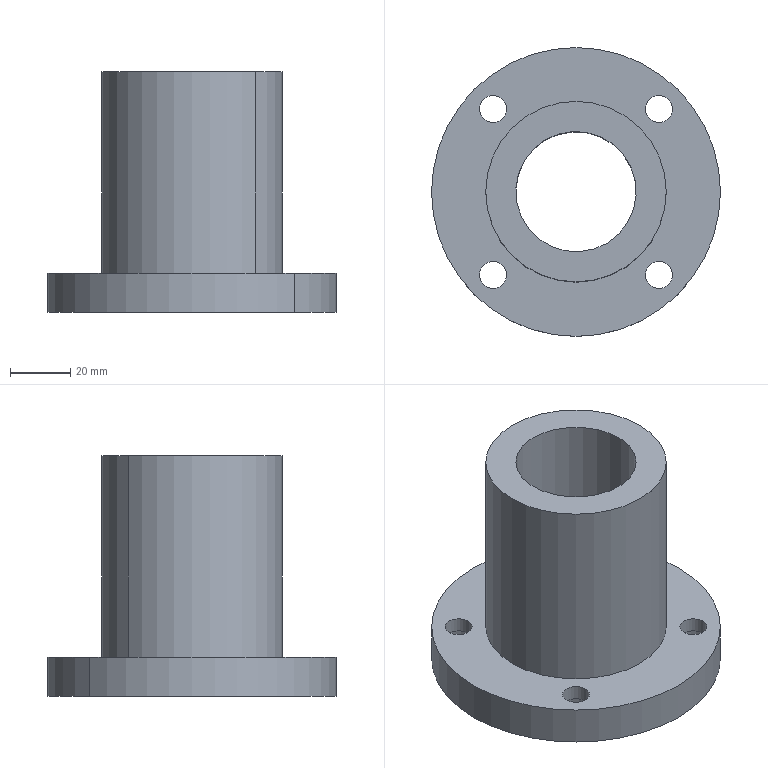Component | SolidWorks | LMF40UU-13 | 1 solid | 29 faces | box 96 x 96 x 80 mm | volume 176770 mm3 | cylinder 22 | plane 7 | commonest cylinder face diameters 9 x8 14 x8 96 x2 40 x2 60 x2 | material Standard Parts
STEP:
#1=CARTESIAN_POINT('',(7.771,5.019,-18.07));
#2=VERTEX_POINT('',#1);
#3=CARTESIAN_POINT('',(7.521,5.269,-18.07));
#4=VERTEX_POINT('',#3);
#5=CARTESIAN_POINT('',(7.646,5.144,-18.07));
#6=DIRECTION('',(0.,0.,-1.));
#7=DIRECTION('',(-0.7071,0.7071,0.));
#8=AXIS2_PLACEMENT_3D('',#5,#6,#7);
#9=CIRCLE('',#8,0.1772);
#10=EDGE_CURVE('',#2,#4,#9,.T.);
#11=ORIENTED_EDGE('',*,*,#10,.F.);
#12=CARTESIAN_POINT('',(7.771,5.019,-18.262));
#13=VERTEX_POINT('',#12);
#14=CARTESIAN_POINT('',(7.771,5.019,-18.262));
#15=DIRECTION('',(0.,0.,-1.));
#16=VECTOR('',#15,39.37);
#17=LINE('',#14,#16);
#18=EDGE_CURVE('',#2,#13,#17,.T.);
#19=ORIENTED_EDGE('',*,*,#18,.T.);
#20=CARTESIAN_POINT('',(7.521,5.269,-18.262));
#21=VERTEX_POINT('',#20);
#22=CARTESIAN_POINT('',(7.646,5.144,-18.262));
#23=DIRECTION('',(0.,0.,-1.));
#24=DIRECTION('',(-0.7071,0.7071,0.));
#25=AXIS2_PLACEMENT_3D('',#22,#23,#24);
#26=CIRCLE('',#25,0.1772);
#27=EDGE_CURVE('',#13,#21,#26,.T.);
#28=ORIENTED_EDGE('',*,*,#27,.T.);
#29=CARTESIAN_POINT('',(7.521,5.269,-18.262));
#30=DIRECTION('',(0.,0.,-1.));
#31=VECTOR('',#30,39.37);
#32=LINE('',#29,#31);
#33=EDGE_CURVE('',#4,#21,#32,.T.);
#34=ORIENTED_EDGE('',*,*,#33,.F.);
#35=EDGE_LOOP('',(#11,#19,#28,#34));
#36=FACE_OUTER_BOUND('',#35,.T.);
#37=CARTESIAN_POINT('',(7.646,5.144,-18.262));
#38=DIRECTION('',(0.,0.,-1.));
#39=DIRECTION('',(-0.7071,0.7071,0.));
#40=AXIS2_PLACEMENT_3D('',#37,#38,#39);
#41=CYLINDRICAL_SURFACE('',#40,0.1772);
#42=ADVANCED_FACE('',(#36),#41,.F.);
#43=CARTESIAN_POINT('',(7.771,2.847,-18.07));
#44=VERTEX_POINT('',#43);
#45=CARTESIAN_POINT('',(7.521,3.098,-18.07));
#46=VERTEX_POINT('',#45);
#47=CARTESIAN_POINT('',(7.646,2.973,-18.07));
#48=DIRECTION('',(0.,0.,-1.));
#49=DIRECTION('',(-0.7071,0.7071,0.));
#50=AXIS2_PLACEMENT_3D('',#47,#48,#49);
#51=CIRCLE('',#50,0.1772);
#52=EDGE_CURVE('',#44,#46,#51,.T.);
#53=ORIENTED_EDGE('',*,*,#52,.F.);
#54=CARTESIAN_POINT('',(7.771,2.847,-18.262));
#55=VERTEX_POINT('',#54);
#56=CARTESIAN_POINT('',(7.771,2.847,-18.262));
#57=DIRECTION('',(0.,0.,-1.));
#58=VECTOR('',#57,39.37);
#59=LINE('',#56,#58);
#60=EDGE_CURVE('',#44,#55,#59,.T.);
#61=ORIENTED_EDGE('',*,*,#60,.T.);
#62=CARTESIAN_POINT('',(7.521,3.098,-18.262));
#63=VERTEX_POINT('',#62);
#64=CARTESIAN_POINT('',(7.646,2.973,-18.262));
#65=DIRECTION('',(0.,0.,-1.));
#66=DIRECTION('',(-0.7071,0.7071,0.));
#67=AXIS2_PLACEMENT_3D('',#64,#65,#66);
#68=CIRCLE('',#67,0.1772);
#69=EDGE_CURVE('',#55,#63,#68,.T.);
#70=ORIENTED_EDGE('',*,*,#69,.T.);
#71=CARTESIAN_POINT('',(7.521,3.098,-18.262));
#72=DIRECTION('',(0.,0.,-1.));
#73=VECTOR('',#72,39.37);
#74=LINE('',#71,#73);
#75=EDGE_CURVE('',#46,#63,#74,.T.);
#76=ORIENTED_EDGE('',*,*,#75,.F.);
#77=EDGE_LOOP('',(#53,#61,#70,#76));
#78=FACE_OUTER_BOUND('',#77,.T.);
#79=CARTESIAN_POINT('',(7.646,2.973,-18.262));
#80=DIRECTION('',(0.,0.,-1.));
#81=DIRECTION('',(-0.7071,0.7071,0.));
#82=AXIS2_PLACEMENT_3D('',#79,#80,#81);
#83=CYLINDRICAL_SURFACE('',#82,0.1772);
#84=ADVANCED_FACE('',(#78),#83,.F.);
#85=CARTESIAN_POINT('',(9.943,2.847,-18.07));
#86=VERTEX_POINT('',#85);
#87=CARTESIAN_POINT('',(9.692,3.098,-18.07));
#88=VERTEX_POINT('',#87);
#89=CARTESIAN_POINT('',(9.817,2.973,-18.07));
#90=DIRECTION('',(0.,0.,-1.));
#91=DIRECTION('',(-0.7071,0.7071,0.));
#92=AXIS2_PLACEMENT_3D('',#89,#90,#91);
#93=CIRCLE('',#92,0.1772);
#94=EDGE_CURVE('',#86,#88,#93,.T.);
#95=ORIENTED_EDGE('',*,*,#94,.F.);
#96=CARTESIAN_POINT('',(9.943,2.847,-18.262));
#97=VERTEX_POINT('',#96);
#98=CARTESIAN_POINT('',(9.943,2.847,-18.262));
#99=DIRECTION('',(0.,0.,-1.));
#100=VECTOR('',#99,39.37);
#101=LINE('',#98,#100);
#102=EDGE_CURVE('',#86,#97,#101,.T.);
#103=ORIENTED_EDGE('',*,*,#102,.T.);
#104=CARTESIAN_POINT('',(9.692,3.098,-18.262));
#105=VERTEX_POINT('',#104);
#106=CARTESIAN_POINT('',(9.817,2.973,-18.262));
#107=DIRECTION('',(0.,0.,-1.));
#108=DIRECTION('',(-0.7071,0.7071,0.));
#109=AXIS2_PLACEMENT_3D('',#106,#107,#108);
#110=CIRCLE('',#109,0.1772);
#111=EDGE_CURVE('',#97,#105,#110,.T.);
#112=ORIENTED_EDGE('',*,*,#111,.T.);
#113=CARTESIAN_POINT('',(9.692,3.098,-18.262));
#114=DIRECTION('',(0.,0.,-1.));
#115=VECTOR('',#114,39.37);
#116=LINE('',#113,#115);
#117=EDGE_CURVE('',#88,#105,#116,.T.);
#118=ORIENTED_EDGE('',*,*,#117,.F.);
#119=EDGE_LOOP('',(#95,#103,#112,#118));
#120=FACE_OUTER_BOUND('',#119,.T.);
#121=CARTESIAN_POINT('',(9.817,2.973,-18.262));
#122=DIRECTION('',(0.,0.,-1.));
#123=DIRECTION('',(-0.7071,0.7071,0.));
#124=AXIS2_PLACEMENT_3D('',#121,#122,#123);
#125=CYLINDRICAL_SURFACE('',#124,0.1772);
#126=ADVANCED_FACE('',(#120),#125,.F.);
#127=CARTESIAN_POINT('',(7.841,4.949,-18.262));
#128=VERTEX_POINT('',#127);
#129=CARTESIAN_POINT('',(7.451,5.339,-18.262));
#130=VERTEX_POINT('',#129);
#131=CARTESIAN_POINT('',(7.646,5.144,-18.262));
#132=DIRECTION('',(0.,0.,-1.));
#133=DIRECTION('',(-0.7071,0.7071,0.));
#134=AXIS2_PLACEMENT_3D('',#131,#132,#133);
#135=CIRCLE('',#134,0.2756);
#136=EDGE_CURVE('',#128,#130,#135,.T.);
#137=ORIENTED_EDGE('',*,*,#136,.F.);
#138=CARTESIAN_POINT('',(7.841,4.949,-18.581));
#139=VERTEX_POINT('',#138);
#140=CARTESIAN_POINT('',(7.841,4.949,-18.581));
#141=DIRECTION('',(0.,0.,-1.));
#142=VECTOR('',#141,39.37);
#143=LINE('',#140,#142);
#144=EDGE_CURVE('',#128,#139,#143,.T.);
#145=ORIENTED_EDGE('',*,*,#144,.T.);
#146=CARTESIAN_POINT('',(7.451,5.339,-18.581));
#147=VERTEX_POINT('',#146);
#148=CARTESIAN_POINT('',(7.646,5.144,-18.581));
#149=DIRECTION('',(0.,0.,-1.));
#150=DIRECTION('',(-0.7071,0.7071,0.));
#151=AXIS2_PLACEMENT_3D('',#148,#149,#150);
#152=CIRCLE('',#151,0.2756);
#153=EDGE_CURVE('',#139,#147,#152,.T.);
#154=ORIENTED_EDGE('',*,*,#153,.T.);
#155=CARTESIAN_POINT('',(7.451,5.339,-18.581));
#156=DIRECTION('',(0.,0.,-1.));
#157=VECTOR('',#156,39.37);
#158=LINE('',#155,#157);
#159=EDGE_CURVE('',#130,#147,#158,.T.);
#160=ORIENTED_EDGE('',*,*,#159,.F.);
#161=EDGE_LOOP('',(#137,#145,#154,#160));
#162=FACE_OUTER_BOUND('',#161,.T.);
#163=CARTESIAN_POINT('',(7.646,5.144,-18.581));
#164=DIRECTION('',(0.,0.,-1.));
#165=DIRECTION('',(-0.7071,0.7071,0.));
#166=AXIS2_PLACEMENT_3D('',#163,#164,#165);
#167=CYLINDRICAL_SURFACE('',#166,0.2756);
#168=ADVANCED_FACE('',(#162),#167,.F.);
#169=CARTESIAN_POINT('',(7.841,2.778,-18.262));
#170=VERTEX_POINT('',#169);
#171=CARTESIAN_POINT('',(7.451,3.168,-18.262));
#172=VERTEX_POINT('',#171);
#173=CARTESIAN_POINT('',(7.646,2.973,-18.262));
#174=DIRECTION('',(0.,0.,-1.));
#175=DIRECTION('',(-0.7071,0.7071,0.));
#176=AXIS2_PLACEMENT_3D('',#173,#174,#175);
#177=CIRCLE('',#176,0.2756);
#178=EDGE_CURVE('',#170,#172,#177,.T.);
#179=ORIENTED_EDGE('',*,*,#178,.F.);
#180=CARTESIAN_POINT('',(7.841,2.778,-18.581));
#181=VERTEX_POINT('',#180);
#182=CARTESIAN_POINT('',(7.841,2.778,-18.581));
#183=DIRECTION('',(0.,0.,-1.));
#184=VECTOR('',#183,39.37);
#185=LINE('',#182,#184);
#186=EDGE_CURVE('',#170,#181,#185,.T.);
#187=ORIENTED_EDGE('',*,*,#186,.T.);
#188=CARTESIAN_POINT('',(7.451,3.168,-18.581));
#189=VERTEX_POINT('',#188);
#190=CARTESIAN_POINT('',(7.646,2.973,-18.581));
#191=DIRECTION('',(0.,0.,-1.));
#192=DIRECTION('',(-0.7071,0.7071,0.));
#193=AXIS2_PLACEMENT_3D('',#190,#191,#192);
#194=CIRCLE('',#193,0.2756);
#195=EDGE_CURVE('',#181,#189,#194,.T.);
#196=ORIENTED_EDGE('',*,*,#195,.T.);
#197=CARTESIAN_POINT('',(7.451,3.168,-18.581));
#198=DIRECTION('',(0.,0.,-1.));
#199=VECTOR('',#198,39.37);
#200=LINE('',#197,#199);
#201=EDGE_CURVE('',#172,#189,#200,.T.);
#202=ORIENTED_EDGE('',*,*,#201,.F.);
#203=EDGE_LOOP('',(#179,#187,#196,#202));
#204=FACE_OUTER_BOUND('',#203,.T.);
#205=CARTESIAN_POINT('',(7.646,2.973,-18.581));
#206=DIRECTION('',(0.,0.,-1.));
#207=DIRECTION('',(-0.7071,0.7071,0.));
#208=AXIS2_PLACEMENT_3D('',#205,#206,#207);
#209=CYLINDRICAL_SURFACE('',#208,0.2756);
#210=ADVANCED_FACE('',(#204),#209,.F.);
#211=CARTESIAN_POINT('',(10.012,2.778,-18.262));
#212=VERTEX_POINT('',#211);
#213=CARTESIAN_POINT('',(9.623,3.168,-18.262));
#214=VERTEX_POINT('',#213);
#215=CARTESIAN_POINT('',(9.817,2.973,-18.262));
#216=DIRECTION('',(0.,0.,-1.));
#217=DIRECTION('',(-0.7071,0.7071,0.));
#218=AXIS2_PLACEMENT_3D('',#215,#216,#217);
#219=CIRCLE('',#218,0.2756);
#220=EDGE_CURVE('',#212,#214,#219,.T.);
#221=ORIENTED_EDGE('',*,*,#220,.F.);
#222=CARTESIAN_POINT('',(10.012,2.778,-18.581));
#223=VERTEX_POINT('',#222);
#224=CARTESIAN_POINT('',(10.012,2.778,-18.581));
#225=DIRECTION('',(0.,0.,-1.));
#226=VECTOR('',#225,39.37);
#227=LINE('',#224,#226);
#228=EDGE_CURVE('',#212,#223,#227,.T.);
#229=ORIENTED_EDGE('',*,*,#228,.T.);
#230=CARTESIAN_POINT('',(9.623,3.168,-18.581));
#231=VERTEX_POINT('',#230);
#232=CARTESIAN_POINT('',(9.817,2.973,-18.581));
#233=DIRECTION('',(0.,0.,-1.));
#234=DIRECTION('',(-0.7071,0.7071,0.));
#235=AXIS2_PLACEMENT_3D('',#232,#233,#234);
#236=CIRCLE('',#235,0.2756);
#237=EDGE_CURVE('',#223,#231,#236,.T.);
#238=ORIENTED_EDGE('',*,*,#237,.T.);
#239=CARTESIAN_POINT('',(9.623,3.168,-18.581));
#240=DIRECTION('',(0.,0.,-1.));
#241=VECTOR('',#240,39.37);
#242=LINE('',#239,#241);
#243=EDGE_CURVE('',#214,#231,#242,.T.);
#244=ORIENTED_EDGE('',*,*,#243,.F.);
#245=EDGE_LOOP('',(#221,#229,#238,#244));
#246=FACE_OUTER_BOUND('',#245,.T.);
#247=CARTESIAN_POINT('',(9.817,2.973,-18.581));
#248=DIRECTION('',(0.,0.,-1.));
#249=DIRECTION('',(-0.7071,0.7071,0.));
#250=AXIS2_PLACEMENT_3D('',#247,#248,#249);
#251=CYLINDRICAL_SURFACE('',#250,0.2756);
#252=ADVANCED_FACE('',(#246),#251,.F.);
#253=CARTESIAN_POINT('',(9.943,5.019,-18.07));
#254=VERTEX_POINT('',#253);
#255=CARTESIAN_POINT('',(9.692,5.269,-18.07));
#256=VERTEX_POINT('',#255);
#257=CARTESIAN_POINT('',(9.817,5.144,-18.07));
#258=DIRECTION('',(0.,0.,-1.));
#259=DIRECTION('',(-0.7071,0.7071,0.));
#260=AXIS2_PLACEMENT_3D('',#257,#258,#259);
#261=CIRCLE('',#260,0.1772);
#262=EDGE_CURVE('',#254,#256,#261,.T.);
#263=ORIENTED_EDGE('',*,*,#262,.F.);
#264=CARTESIAN_POINT('',(9.943,5.019,-18.262));
#265=VERTEX_POINT('',#264);
#266=CARTESIAN_POINT('',(9.943,5.019,-18.262));
#267=DIRECTION('',(0.,0.,-1.));
#268=VECTOR('',#267,39.37);
#269=LINE('',#266,#268);
#270=EDGE_CURVE('',#254,#265,#269,.T.);
#271=ORIENTED_EDGE('',*,*,#270,.T.);
#272=CARTESIAN_POINT('',(9.692,5.269,-18.262));
#273=VERTEX_POINT('',#272);
#274=CARTESIAN_POINT('',(9.817,5.144,-18.262));
#275=DIRECTION('',(0.,0.,-1.));
#276=DIRECTION('',(-0.7071,0.7071,0.));
#277=AXIS2_PLACEMENT_3D('',#274,#275,#276);
#278=CIRCLE('',#277,0.1772);
#279=EDGE_CURVE('',#265,#273,#278,.T.);
#280=ORIENTED_EDGE('',*,*,#279,.T.);
#281=CARTESIAN_POINT('',(9.692,5.269,-18.262));
#282=DIRECTION('',(0.,0.,-1.));
#283=VECTOR('',#282,39.37);
#284=LINE('',#281,#283);
#285=EDGE_CURVE('',#256,#273,#284,.T.);
#286=ORIENTED_EDGE('',*,*,#285,.F.);
#287=EDGE_LOOP('',(#263,#271,#280,#286));
#288=FACE_OUTER_BOUND('',#287,.T.);
#289=CARTESIAN_POINT('',(9.817,5.144,-18.262));
#290=DIRECTION('',(0.,0.,-1.));
#291=DIRECTION('',(-0.7071,0.7071,0.));
#292=AXIS2_PLACEMENT_3D('',#289,#290,#291);
#293=CYLINDRICAL_SURFACE('',#292,0.1772);
#294=ADVANCED_FACE('',(#288),#293,.F.);
#295=CARTESIAN_POINT('',(10.012,4.949,-18.262));
#296=VERTEX_POINT('',#295);
#297=CARTESIAN_POINT('',(9.623,5.339,-18.262));
#298=VERTEX_POINT('',#297);
#299=CARTESIAN_POINT('',(9.817,5.144,-18.262));
#300=DIRECTION('',(0.,0.,-1.));
#301=DIRECTION('',(-0.7071,0.7071,0.));
#302=AXIS2_PLACEMENT_3D('',#299,#300,#301);
#303=CIRCLE('',#302,0.2756);
#304=EDGE_CURVE('',#296,#298,#303,.T.);
#305=ORIENTED_EDGE('',*,*,#304,.F.);
#306=CARTESIAN_POINT('',(10.012,4.949,-18.581));
#307=VERTEX_POINT('',#306);
#308=CARTESIAN_POINT('',(10.012,4.949,-18.581));
#309=DIRECTION('',(0.,0.,-1.));
#310=VECTOR('',#309,39.37);
#311=LINE('',#308,#310);
#312=EDGE_CURVE('',#296,#307,#311,.T.);
#313=ORIENTED_EDGE('',*,*,#312,.T.);
#314=CARTESIAN_POINT('',(9.623,5.339,-18.581));
#315=VERTEX_POINT('',#314);
#316=CARTESIAN_POINT('',(9.817,5.144,-18.581));
#317=DIRECTION('',(0.,0.,-1.));
#318=DIRECTION('',(-0.7071,0.7071,0.));
#319=AXIS2_PLACEMENT_3D('',#316,#317,#318);
#320=CIRCLE('',#319,0.2756);
#321=EDGE_CURVE('',#307,#315,#320,.T.);
#322=ORIENTED_EDGE('',*,*,#321,.T.);
#323=CARTESIAN_POINT('',(9.623,5.339,-18.581));
#324=DIRECTION('',(0.,0.,-1.));
#325=VECTOR('',#324,39.37);
#326=LINE('',#323,#325);
#327=EDGE_CURVE('',#298,#315,#326,.T.);
#328=ORIENTED_EDGE('',*,*,#327,.F.);
#329=EDGE_LOOP('',(#305,#313,#322,#328));
#330=FACE_OUTER_BOUND('',#329,.T.);
#331=CARTESIAN_POINT('',(9.817,5.144,-18.581));
#332=DIRECTION('',(0.,0.,-1.));
#333=DIRECTION('',(-0.7071,0.7071,0.));
#334=AXIS2_PLACEMENT_3D('',#331,#332,#333);
#335=CYLINDRICAL_SURFACE('',#334,0.2756);
#336=ADVANCED_FACE('',(#330),#335,.F.);
#337=CARTESIAN_POINT('',(7.395,5.395,-18.07));
#338=VERTEX_POINT('',#337);
#339=CARTESIAN_POINT('',(10.068,2.722,-18.07));
#340=VERTEX_POINT('',#339);
#341=CARTESIAN_POINT('',(8.732,4.058,-18.07));
#342=DIRECTION('',(0.,0.,-1.));
#343=DIRECTION('',(-0.7071,0.7071,0.));
#344=AXIS2_PLACEMENT_3D('',#341,#342,#343);
#345=CIRCLE('',#344,1.89);
#346=EDGE_CURVE('',#338,#340,#345,.T.);
#347=ORIENTED_EDGE('',*,*,#346,.T.);
#348=CARTESIAN_POINT('',(10.068,2.722,-18.581));
#349=VERTEX_POINT('',#348);
#350=CARTESIAN_POINT('',(10.068,2.722,-18.07));
#351=DIRECTION('',(0.,0.,-1.));
#352=VECTOR('',#351,39.37);
#353=LINE('',#350,#352);
#354=EDGE_CURVE('',#340,#349,#353,.T.);
#355=ORIENTED_EDGE('',*,*,#354,.T.);
#356=CARTESIAN_POINT('',(7.395,5.395,-18.581));
#357=VERTEX_POINT('',#356);
#358=CARTESIAN_POINT('',(8.732,4.058,-18.581));
#359=DIRECTION('',(0.,0.,-1.));
#360=DIRECTION('',(-0.7071,0.7071,0.));
#361=AXIS2_PLACEMENT_3D('',#358,#359,#360);
#362=CIRCLE('',#361,1.89);
#363=EDGE_CURVE('',#357,#349,#362,.T.);
#364=ORIENTED_EDGE('',*,*,#363,.F.);
#365=CARTESIAN_POINT('',(7.395,5.395,-18.07));
#366=DIRECTION('',(0.,0.,-1.));
#367=VECTOR('',#366,39.37);
#368=LINE('',#365,#367);
#369=EDGE_CURVE('',#338,#357,#368,.T.);
#370=ORIENTED_EDGE('',*,*,#369,.F.);
#371=EDGE_LOOP('',(#347,#355,#364,#370));
#372=FACE_OUTER_BOUND('',#371,.T.);
#373=CARTESIAN_POINT('',(8.732,4.058,-18.07));
#374=DIRECTION('',(0.,0.,-1.));
#375=DIRECTION('',(-0.7071,0.7071,0.));
#376=AXIS2_PLACEMENT_3D('',#373,#374,#375);
#377=CYLINDRICAL_SURFACE('',#376,1.89);
#378=ADVANCED_FACE('',(#372),#377,.T.);
#379=CARTESIAN_POINT('',(9.288,3.502,-15.432));
#380=VERTEX_POINT('',#379);
#381=CARTESIAN_POINT('',(8.175,4.615,-15.432));
#382=VERTEX_POINT('',#381);
#383=CARTESIAN_POINT('',(8.732,4.058,-15.432));
#384=DIRECTION('',(0.,0.,-1.));
#385=DIRECTION('',(-0.7071,0.7071,0.));
#386=AXIS2_PLACEMENT_3D('',#383,#384,#385);
#387=CIRCLE('',#386,0.7874);
#388=EDGE_CURVE('',#380,#382,#387,.T.);
#389=ORIENTED_EDGE('',*,*,#388,.F.);
#390=CARTESIAN_POINT('',(9.288,3.502,-18.581));
#391=VERTEX_POINT('',#390);
#392=CARTESIAN_POINT('',(9.288,3.502,-15.432));
#393=DIRECTION('',(0.,0.,-1.));
#394=VECTOR('',#393,39.37);
#395=LINE('',#392,#394);
#396=EDGE_CURVE('',#380,#391,#395,.T.);
#397=ORIENTED_EDGE('',*,*,#396,.T.);
#398=CARTESIAN_POINT('',(8.175,4.615,-18.581));
#399=VERTEX_POINT('',#398);
#400=CARTESIAN_POINT('',(8.732,4.058,-18.581));
#401=DIRECTION('',(0.,0.,-1.));
#402=DIRECTION('',(-0.7071,0.7071,0.));
#403=AXIS2_PLACEMENT_3D('',#400,#401,#402);
#404=CIRCLE('',#403,0.7874);
#405=EDGE_CURVE('',#391,#399,#404,.T.);
#406=ORIENTED_EDGE('',*,*,#405,.T.);
#407=CARTESIAN_POINT('',(8.175,4.615,-15.432));
#408=DIRECTION('',(0.,0.,-1.));
#409=VECTOR('',#408,39.37);
#410=LINE('',#407,#409);
#411=EDGE_CURVE('',#382,#399,#410,.T.);
#412=ORIENTED_EDGE('',*,*,#411,.F.);
#413=EDGE_LOOP('',(#389,#397,#406,#412));
#414=FACE_OUTER_BOUND('',#413,.T.);
#415=CARTESIAN_POINT('',(8.732,4.058,-15.432));
#416=DIRECTION('',(0.,0.,-1.));
#417=DIRECTION('',(-0.7071,0.7071,0.));
#418=AXIS2_PLACEMENT_3D('',#415,#416,#417);
#419=CYLINDRICAL_SURFACE('',#418,0.7874);
#420=ADVANCED_FACE('',(#414),#419,.F.);
#421=CARTESIAN_POINT('',(7.897,4.894,-15.432));
#422=VERTEX_POINT('',#421);
#423=CARTESIAN_POINT('',(9.567,3.223,-15.432));
#424=VERTEX_POINT('',#423);
#425=CARTESIAN_POINT('',(8.732,4.058,-15.432));
#426=DIRECTION('',(0.,0.,-1.));
#427=DIRECTION('',(-0.7071,0.7071,0.));
#428=AXIS2_PLACEMENT_3D('',#425,#426,#427);
#429=CIRCLE('',#428,1.181);
#430=EDGE_CURVE('',#422,#424,#429,.T.);
#431=ORIENTED_EDGE('',*,*,#430,.T.);
#432=CARTESIAN_POINT('',(9.567,3.223,-18.07));
#433=VERTEX_POINT('',#432);
#434=CARTESIAN_POINT('',(9.567,3.223,-15.432));
#435=DIRECTION('',(0.,0.,-1.));
#436=VECTOR('',#435,39.37);
#437=LINE('',#434,#436);
#438=EDGE_CURVE('',#424,#433,#437,.T.);
#439=ORIENTED_EDGE('',*,*,#438,.T.);
#440=CARTESIAN_POINT('',(7.897,4.894,-18.07));
#441=VERTEX_POINT('',#440);
#442=CARTESIAN_POINT('',(8.732,4.058,-18.07));
#443=DIRECTION('',(0.,0.,1.));
#444=DIRECTION('',(-0.7071,0.7071,0.));
#445=AXIS2_PLACEMENT_3D('',#442,#443,#444);
#446=CIRCLE('',#445,1.181);
#447=EDGE_CURVE('',#433,#441,#446,.T.);
#448=ORIENTED_EDGE('',*,*,#447,.T.);
#449=CARTESIAN_POINT('',(7.897,4.894,-15.432));
#450=DIRECTION('',(0.,0.,-1.));
#451=VECTOR('',#450,39.37);
#452=LINE('',#449,#451);
#453=EDGE_CURVE('',#422,#441,#452,.T.);
#454=ORIENTED_EDGE('',*,*,#453,.F.);
#455=EDGE_LOOP('',(#431,#439,#448,#454));
#456=FACE_OUTER_BOUND('',#455,.T.);
#457=CARTESIAN_POINT('',(8.732,4.058,-15.432));
#458=DIRECTION('',(0.,0.,-1.));
#459=DIRECTION('',(-0.7071,0.7071,0.));
#460=AXIS2_PLACEMENT_3D('',#457,#458,#459);
#461=CYLINDRICAL_SURFACE('',#460,1.181);
#462=ADVANCED_FACE('',(#456),#461,.T.);
#463=CARTESIAN_POINT('',(7.646,5.144,-18.262));
#464=DIRECTION('',(0.,0.,-1.));
#465=DIRECTION('',(-0.7071,0.7071,0.));
#466=AXIS2_PLACEMENT_3D('',#463,#464,#465);
#467=CIRCLE('',#466,0.2756);
#468=EDGE_CURVE('',#130,#128,#467,.T.);
#469=ORIENTED_EDGE('',*,*,#468,.T.);
#470=ORIENTED_EDGE('',*,*,#136,.T.);
#471=EDGE_LOOP('',(#469,#470));
#472=FACE_OUTER_BOUND('',#471,.T.);
#473=CARTESIAN_POINT('',(7.646,5.144,-18.262));
#474=DIRECTION('',(0.,0.,-1.));
#475=DIRECTION('',(-0.7071,0.7071,0.));
#476=AXIS2_PLACEMENT_3D('',#473,#474,#475);
#477=CIRCLE('',#476,0.1772);
#478=EDGE_CURVE('',#21,#13,#477,.T.);
#479=ORIENTED_EDGE('',*,*,#478,.F.);
#480=ORIENTED_EDGE('',*,*,#27,.F.);
#481=EDGE_LOOP('',(#479,#480));
#482=FACE_BOUND('',#481,.T.);
#483=CARTESIAN_POINT('',(7.646,5.144,-18.262));
#484=DIRECTION('',(0.,0.,1.));
#485=DIRECTION('',(0.7071,-0.7071,0.));
#486=AXIS2_PLACEMENT_3D('',#483,#484,#485);
#487=PLANE('',#486);
#488=ADVANCED_FACE('',(#472,#482),#487,.F.);
#489=CARTESIAN_POINT('',(7.646,2.973,-18.262));
#490=DIRECTION('',(0.,0.,-1.));
#491=DIRECTION('',(-0.7071,0.7071,0.));
#492=AXIS2_PLACEMENT_3D('',#489,#490,#491);
#493=CIRCLE('',#492,0.2756);
#494=EDGE_CURVE('',#172,#170,#493,.T.);
#495=ORIENTED_EDGE('',*,*,#494,.T.);
#496=ORIENTED_EDGE('',*,*,#178,.T.);
#497=EDGE_LOOP('',(#495,#496));
#498=FACE_OUTER_BOUND('',#497,.T.);
#499=CARTESIAN_POINT('',(7.646,2.973,-18.262));
#500=DIRECTION('',(0.,0.,-1.));
#501=DIRECTION('',(-0.7071,0.7071,0.));
#502=AXIS2_PLACEMENT_3D('',#499,#500,#501);
#503=CIRCLE('',#502,0.1772);
#504=EDGE_CURVE('',#63,#55,#503,.T.);
#505=ORIENTED_EDGE('',*,*,#504,.F.);
#506=ORIENTED_EDGE('',*,*,#69,.F.);
#507=EDGE_LOOP('',(#505,#506));
#508=FACE_BOUND('',#507,.T.);
#509=CARTESIAN_POINT('',(7.646,2.973,-18.262));
#510=DIRECTION('',(0.,0.,1.));
#511=DIRECTION('',(0.7071,-0.7071,0.));
#512=AXIS2_PLACEMENT_3D('',#509,#510,#511);
#513=PLANE('',#512);
#514=ADVANCED_FACE('',(#498,#508),#513,.F.);
#515=CARTESIAN_POINT('',(9.817,2.973,-18.262));
#516=DIRECTION('',(0.,0.,-1.));
#517=DIRECTION('',(-0.7071,0.7071,0.));
#518=AXIS2_PLACEMENT_3D('',#515,#516,#517);
#519=CIRCLE('',#518,0.2756);
#520=EDGE_CURVE('',#214,#212,#519,.T.);
#521=ORIENTED_EDGE('',*,*,#520,.T.);
#522=ORIENTED_EDGE('',*,*,#220,.T.);
#523=EDGE_LOOP('',(#521,#522));
#524=FACE_OUTER_BOUND('',#523,.T.);
#525=CARTESIAN_POINT('',(9.817,2.973,-18.262));
#526=DIRECTION('',(0.,0.,-1.));
#527=DIRECTION('',(-0.7071,0.7071,0.));
#528=AXIS2_PLACEMENT_3D('',#525,#526,#527);
#529=CIRCLE('',#528,0.1772);
#530=EDGE_CURVE('',#105,#97,#529,.T.);
#531=ORIENTED_EDGE('',*,*,#530,.F.);
#532=ORIENTED_EDGE('',*,*,#111,.F.);
#533=EDGE_LOOP('',(#531,#532));
#534=FACE_BOUND('',#533,.T.);
#535=CARTESIAN_POINT('',(9.817,2.973,-18.262));
#536=DIRECTION('',(0.,0.,1.));
#537=DIRECTION('',(0.7071,-0.7071,0.));
#538=AXIS2_PLACEMENT_3D('',#535,#536,#537);
#539=PLANE('',#538);
#540=ADVANCED_FACE('',(#524,#534),#539,.F.);
#541=CARTESIAN_POINT('',(9.817,5.144,-18.262));
#542=DIRECTION('',(0.,0.,-1.));
#543=DIRECTION('',(-0.7071,0.7071,0.));
#544=AXIS2_PLACEMENT_3D('',#541,#542,#543);
#545=CIRCLE('',#544,0.2756);
#546=EDGE_CURVE('',#298,#296,#545,.T.);
#547=ORIENTED_EDGE('',*,*,#546,.T.);
#548=ORIENTED_EDGE('',*,*,#304,.T.);
#549=EDGE_LOOP('',(#547,#548));
#550=FACE_OUTER_BOUND('',#549,.T.);
#551=CARTESIAN_POINT('',(9.817,5.144,-18.262));
#552=DIRECTION('',(0.,0.,-1.));
#553=DIRECTION('',(-0.7071,0.7071,0.));
#554=AXIS2_PLACEMENT_3D('',#551,#552,#553);
#555=CIRCLE('',#554,0.1772);
#556=EDGE_CURVE('',#273,#265,#555,.T.);
#557=ORIENTED_EDGE('',*,*,#556,.F.);
#558=ORIENTED_EDGE('',*,*,#279,.F.);
#559=EDGE_LOOP('',(#557,#558));
#560=FACE_BOUND('',#559,.T.);
#561=CARTESIAN_POINT('',(9.817,5.144,-18.262));
#562=DIRECTION('',(0.,0.,1.));
#563=DIRECTION('',(0.7071,-0.7071,0.));
#564=AXIS2_PLACEMENT_3D('',#561,#562,#563);
#565=PLANE('',#564);
#566=ADVANCED_FACE('',(#550,#560),#565,.F.);
#567=ORIENTED_EDGE('',*,*,#438,.F.);
#568=CARTESIAN_POINT('',(8.732,4.058,-15.432));
#569=DIRECTION('',(0.,0.,-1.));
#570=DIRECTION('',(-0.7071,0.7071,0.));
#571=AXIS2_PLACEMENT_3D('',#568,#569,#570);
#572=CIRCLE('',#571,1.181);
#573=EDGE_CURVE('',#424,#422,#572,.T.);
#574=ORIENTED_EDGE('',*,*,#573,.T.);
#575=ORIENTED_EDGE('',*,*,#453,.T.);
#576=CARTESIAN_POINT('',(8.732,4.058,-18.07));
#577=DIRECTION('',(0.,0.,1.));
#578=DIRECTION('',(-0.7071,0.7071,0.));
#579=AXIS2_PLACEMENT_3D('',#576,#577,#578);
#580=CIRCLE('',#579,1.181);
#581=EDGE_CURVE('',#441,#433,#580,.T.);
#582=ORIENTED_EDGE('',*,*,#581,.T.);
#583=EDGE_LOOP('',(#567,#574,#575,#582));
#584=FACE_OUTER_BOUND('',#583,.T.);
#585=CARTESIAN_POINT('',(8.732,4.058,-15.432));
#586=DIRECTION('',(0.,0.,-1.));
#587=DIRECTION('',(-0.7071,0.7071,0.));
#588=AXIS2_PLACEMENT_3D('',#585,#586,#587);
#589=CYLINDRICAL_SURFACE('',#588,1.181);
#590=ADVANCED_FACE('',(#584),#589,.T.);
#591=CARTESIAN_POINT('',(8.732,4.058,-15.432));
#592=DIRECTION('',(0.,0.,-1.));
#593=DIRECTION('',(-0.7071,0.7071,0.));
#594=AXIS2_PLACEMENT_3D('',#591,#592,#593);
#595=CIRCLE('',#594,0.7874);
#596=EDGE_CURVE('',#382,#380,#595,.T.);
#597=ORIENTED_EDGE('',*,*,#596,.T.);
#598=ORIENTED_EDGE('',*,*,#388,.T.);
#599=EDGE_LOOP('',(#597,#598));
#600=FACE_BOUND('',#599,.T.);
#601=ORIENTED_EDGE('',*,*,#430,.F.);
#602=ORIENTED_EDGE('',*,*,#573,.F.);
#603=EDGE_LOOP('',(#601,#602));
#604=FACE_OUTER_BOUND('',#603,.T.);
#605=CARTESIAN_POINT('',(8.732,4.058,-15.432));
#606=DIRECTION('',(0.,0.,-1.));
#607=DIRECTION('',(-0.7071,0.7071,0.));
#608=AXIS2_PLACEMENT_3D('',#605,#606,#607);
#609=PLANE('',#608);
#610=ADVANCED_FACE('',(#600,#604),#609,.F.);
#611=ORIENTED_EDGE('',*,*,#396,.F.);
#612=ORIENTED_EDGE('',*,*,#596,.F.);
#613=ORIENTED_EDGE('',*,*,#411,.T.);
#614=CARTESIAN_POINT('',(8.732,4.058,-18.581));
#615=DIRECTION('',(0.,0.,-1.));
#616=DIRECTION('',(-0.7071,0.7071,0.));
#617=AXIS2_PLACEMENT_3D('',#614,#615,#616);
#618=CIRCLE('',#617,0.7874);
#619=EDGE_CURVE('',#399,#391,#618,.T.);
#620=ORIENTED_EDGE('',*,*,#619,.T.);
#621=EDGE_LOOP('',(#611,#612,#613,#620));
#622=FACE_OUTER_BOUND('',#621,.T.);
#623=CARTESIAN_POINT('',(8.732,4.058,-15.432));
#624=DIRECTION('',(0.,0.,-1.));
#625=DIRECTION('',(-0.7071,0.7071,0.));
#626=AXIS2_PLACEMENT_3D('',#623,#624,#625);
#627=CYLINDRICAL_SURFACE('',#626,0.7874);
#628=ADVANCED_FACE('',(#622),#627,.F.);
#629=CARTESIAN_POINT('',(7.646,5.144,-18.581));
#630=DIRECTION('',(0.,0.,-1.));
#631=DIRECTION('',(-0.7071,0.7071,0.));
#632=AXIS2_PLACEMENT_3D('',#629,#630,#631);
#633=CIRCLE('',#632,0.2756);
#634=EDGE_CURVE('',#147,#139,#633,.T.);
#635=ORIENTED_EDGE('',*,*,#634,.F.);
#636=ORIENTED_EDGE('',*,*,#153,.F.);
#637=EDGE_LOOP('',(#635,#636));
#638=FACE_BOUND('',#637,.T.);
#639=CARTESIAN_POINT('',(7.646,2.973,-18.581));
#640=DIRECTION('',(0.,0.,-1.));
#641=DIRECTION('',(-0.7071,0.7071,0.));
#642=AXIS2_PLACEMENT_3D('',#639,#640,#641);
#643=CIRCLE('',#642,0.2756);
#644=EDGE_CURVE('',#189,#181,#643,.T.);
#645=ORIENTED_EDGE('',*,*,#644,.F.);
#646=ORIENTED_EDGE('',*,*,#195,.F.);
#647=EDGE_LOOP('',(#645,#646));
#648=FACE_BOUND('',#647,.T.);
#649=CARTESIAN_POINT('',(9.817,2.973,-18.581));
#650=DIRECTION('',(0.,0.,-1.));
#651=DIRECTION('',(-0.7071,0.7071,0.));
#652=AXIS2_PLACEMENT_3D('',#649,#650,#651);
#653=CIRCLE('',#652,0.2756);
#654=EDGE_CURVE('',#231,#223,#653,.T.);
#655=ORIENTED_EDGE('',*,*,#654,.F.);
#656=ORIENTED_EDGE('',*,*,#237,.F.);
#657=EDGE_LOOP('',(#655,#656));
#658=FACE_BOUND('',#657,.T.);
#659=CARTESIAN_POINT('',(9.817,5.144,-18.581));
#660=DIRECTION('',(0.,0.,-1.));
#661=DIRECTION('',(-0.7071,0.7071,0.));
#662=AXIS2_PLACEMENT_3D('',#659,#660,#661);
#663=CIRCLE('',#662,0.2756);
#664=EDGE_CURVE('',#315,#307,#663,.T.);
#665=ORIENTED_EDGE('',*,*,#664,.F.);
#666=ORIENTED_EDGE('',*,*,#321,.F.);
#667=EDGE_LOOP('',(#665,#666));
#668=FACE_BOUND('',#667,.T.);
#669=ORIENTED_EDGE('',*,*,#619,.F.);
#670=ORIENTED_EDGE('',*,*,#405,.F.);
#671=EDGE_LOOP('',(#669,#670));
#672=FACE_BOUND('',#671,.T.);
#673=ORIENTED_EDGE('',*,*,#363,.T.);
#674=CARTESIAN_POINT('',(8.732,4.058,-18.581));
#675=DIRECTION('',(0.,0.,-1.));
#676=DIRECTION('',(-0.7071,0.7071,0.));
#677=AXIS2_PLACEMENT_3D('',#674,#675,#676);
#678=CIRCLE('',#677,1.89);
#679=EDGE_CURVE('',#349,#357,#678,.T.);
#680=ORIENTED_EDGE('',*,*,#679,.T.);
#681=EDGE_LOOP('',(#673,#680));
#682=FACE_OUTER_BOUND('',#681,.T.);
#683=CARTESIAN_POINT('',(8.732,4.058,-18.581));
#684=DIRECTION('',(0.,0.,-1.));
#685=DIRECTION('',(-0.7071,0.7071,0.));
#686=AXIS2_PLACEMENT_3D('',#683,#684,#685);
#687=PLANE('',#686);
#688=ADVANCED_FACE('',(#638,#648,#658,#668,#672,#682),#687,.T.);
#689=ORIENTED_EDGE('',*,*,#354,.F.);
#690=CARTESIAN_POINT('',(8.732,4.058,-18.07));
#691=DIRECTION('',(0.,0.,-1.));
#692=DIRECTION('',(-0.7071,0.7071,0.));
#693=AXIS2_PLACEMENT_3D('',#690,#691,#692);
#694=CIRCLE('',#693,1.89);
#695=EDGE_CURVE('',#340,#338,#694,.T.);
#696=ORIENTED_EDGE('',*,*,#695,.T.);
#697=ORIENTED_EDGE('',*,*,#369,.T.);
#698=ORIENTED_EDGE('',*,*,#679,.F.);
#699=EDGE_LOOP('',(#689,#696,#697,#698));
#700=FACE_OUTER_BOUND('',#699,.T.);
#701=CARTESIAN_POINT('',(8.732,4.058,-18.07));
#702=DIRECTION('',(0.,0.,-1.));
#703=DIRECTION('',(-0.7071,0.7071,0.));
#704=AXIS2_PLACEMENT_3D('',#701,#702,#703);
#705=CYLINDRICAL_SURFACE('',#704,1.89);
#706=ADVANCED_FACE('',(#700),#705,.T.);
#707=CARTESIAN_POINT('',(7.646,5.144,-18.07));
#708=DIRECTION('',(0.,0.,-1.));
#709=DIRECTION('',(-0.7071,0.7071,0.));
#710=AXIS2_PLACEMENT_3D('',#707,#708,#709);
#711=CIRCLE('',#710,0.1772);
#712=EDGE_CURVE('',#4,#2,#711,.T.);
#713=ORIENTED_EDGE('',*,*,#712,.T.);
#714=ORIENTED_EDGE('',*,*,#10,.T.);
#715=EDGE_LOOP('',(#713,#714));
#716=FACE_BOUND('',#715,.T.);
#717=CARTESIAN_POINT('',(7.646,2.973,-18.07));
#718=DIRECTION('',(0.,0.,-1.));
#719=DIRECTION('',(-0.7071,0.7071,0.));
#720=AXIS2_PLACEMENT_3D('',#717,#718,#719);
#721=CIRCLE('',#720,0.1772);
#722=EDGE_CURVE('',#46,#44,#721,.T.);
#723=ORIENTED_EDGE('',*,*,#722,.T.);
#724=ORIENTED_EDGE('',*,*,#52,.T.);
#725=EDGE_LOOP('',(#723,#724));
#726=FACE_BOUND('',#725,.T.);
#727=CARTESIAN_POINT('',(9.817,2.973,-18.07));
#728=DIRECTION('',(0.,0.,-1.));
#729=DIRECTION('',(-0.7071,0.7071,0.));
#730=AXIS2_PLACEMENT_3D('',#727,#728,#729);
#731=CIRCLE('',#730,0.1772);
#732=EDGE_CURVE('',#88,#86,#731,.T.);
#733=ORIENTED_EDGE('',*,*,#732,.T.);
#734=ORIENTED_EDGE('',*,*,#94,.T.);
#735=EDGE_LOOP('',(#733,#734));
#736=FACE_BOUND('',#735,.T.);
#737=CARTESIAN_POINT('',(9.817,5.144,-18.07));
#738=DIRECTION('',(0.,0.,-1.));
#739=DIRECTION('',(-0.7071,0.7071,0.));
#740=AXIS2_PLACEMENT_3D('',#737,#738,#739);
#741=CIRCLE('',#740,0.1772);
#742=EDGE_CURVE('',#256,#254,#741,.T.);
#743=ORIENTED_EDGE('',*,*,#742,.T.);
#744=ORIENTED_EDGE('',*,*,#262,.T.);
#745=EDGE_LOOP('',(#743,#744));
#746=FACE_BOUND('',#745,.T.);
#747=ORIENTED_EDGE('',*,*,#581,.F.);
#748=ORIENTED_EDGE('',*,*,#447,.F.);
#749=EDGE_LOOP('',(#747,#748));
#750=FACE_BOUND('',#749,.T.);
#751=ORIENTED_EDGE('',*,*,#346,.F.);
#752=ORIENTED_EDGE('',*,*,#695,.F.);
#753=EDGE_LOOP('',(#751,#752));
#754=FACE_OUTER_BOUND('',#753,.T.);
#755=CARTESIAN_POINT('',(8.732,4.058,-18.07));
#756=DIRECTION('',(0.,0.,-1.));
#757=DIRECTION('',(-0.7071,0.7071,0.));
#758=AXIS2_PLACEMENT_3D('',#755,#756,#757);
#759=PLANE('',#758);
#760=ADVANCED_FACE('',(#716,#726,#736,#746,#750,#754),#759,.F.);
#761=ORIENTED_EDGE('',*,*,#312,.F.);
#762=ORIENTED_EDGE('',*,*,#546,.F.);
#763=ORIENTED_EDGE('',*,*,#327,.T.);
#764=ORIENTED_EDGE('',*,*,#664,.T.);
#765=EDGE_LOOP('',(#761,#762,#763,#764));
#766=FACE_OUTER_BOUND('',#765,.T.);
#767=CARTESIAN_POINT('',(9.817,5.144,-18.581));
#768=DIRECTION('',(0.,0.,-1.));
#769=DIRECTION('',(-0.7071,0.7071,0.));
#770=AXIS2_PLACEMENT_3D('',#767,#768,#769);
#771=CYLINDRICAL_SURFACE('',#770,0.2756);
#772=ADVANCED_FACE('',(#766),#771,.F.);
#773=ORIENTED_EDGE('',*,*,#270,.F.);
#774=ORIENTED_EDGE('',*,*,#742,.F.);
#775=ORIENTED_EDGE('',*,*,#285,.T.);
#776=ORIENTED_EDGE('',*,*,#556,.T.);
#777=EDGE_LOOP('',(#773,#774,#775,#776));
#778=FACE_OUTER_BOUND('',#777,.T.);
#779=CARTESIAN_POINT('',(9.817,5.144,-18.262));
#780=DIRECTION('',(0.,0.,-1.));
#781=DIRECTION('',(-0.7071,0.7071,0.));
#782=AXIS2_PLACEMENT_3D('',#779,#780,#781);
#783=CYLINDRICAL_SURFACE('',#782,0.1772);
#784=ADVANCED_FACE('',(#778),#783,.F.);
#785=ORIENTED_EDGE('',*,*,#228,.F.);
#786=ORIENTED_EDGE('',*,*,#520,.F.);
#787=ORIENTED_EDGE('',*,*,#243,.T.);
#788=ORIENTED_EDGE('',*,*,#654,.T.);
#789=EDGE_LOOP('',(#785,#786,#787,#788));
#790=FACE_OUTER_BOUND('',#789,.T.);
#791=CARTESIAN_POINT('',(9.817,2.973,-18.581));
#792=DIRECTION('',(0.,0.,-1.));
#793=DIRECTION('',(-0.7071,0.7071,0.));
#794=AXIS2_PLACEMENT_3D('',#791,#792,#793);
#795=CYLINDRICAL_SURFACE('',#794,0.2756);
#796=ADVANCED_FACE('',(#790),#795,.F.);
#797=ORIENTED_EDGE('',*,*,#186,.F.);
#798=ORIENTED_EDGE('',*,*,#494,.F.);
#799=ORIENTED_EDGE('',*,*,#201,.T.);
#800=ORIENTED_EDGE('',*,*,#644,.T.);
#801=EDGE_LOOP('',(#797,#798,#799,#800));
#802=FACE_OUTER_BOUND('',#801,.T.);
#803=CARTESIAN_POINT('',(7.646,2.973,-18.581));
#804=DIRECTION('',(0.,0.,-1.));
#805=DIRECTION('',(-0.7071,0.7071,0.));
#806=AXIS2_PLACEMENT_3D('',#803,#804,#805);
#807=CYLINDRICAL_SURFACE('',#806,0.2756);
#808=ADVANCED_FACE('',(#802),#807,.F.);
#809=ORIENTED_EDGE('',*,*,#144,.F.);
#810=ORIENTED_EDGE('',*,*,#468,.F.);
#811=ORIENTED_EDGE('',*,*,#159,.T.);
#812=ORIENTED_EDGE('',*,*,#634,.T.);
#813=EDGE_LOOP('',(#809,#810,#811,#812));
#814=FACE_OUTER_BOUND('',#813,.T.);
#815=CARTESIAN_POINT('',(7.646,5.144,-18.581));
#816=DIRECTION('',(0.,0.,-1.));
#817=DIRECTION('',(-0.7071,0.7071,0.));
#818=AXIS2_PLACEMENT_3D('',#815,#816,#817);
#819=CYLINDRICAL_SURFACE('',#818,0.2756);
#820=ADVANCED_FACE('',(#814),#819,.F.);
#821=ORIENTED_EDGE('',*,*,#102,.F.);
#822=ORIENTED_EDGE('',*,*,#732,.F.);
#823=ORIENTED_EDGE('',*,*,#117,.T.);
#824=ORIENTED_EDGE('',*,*,#530,.T.);
#825=EDGE_LOOP('',(#821,#822,#823,#824));
#826=FACE_OUTER_BOUND('',#825,.T.);
#827=CARTESIAN_POINT('',(9.817,2.973,-18.262));
#828=DIRECTION('',(0.,0.,-1.));
#829=DIRECTION('',(-0.7071,0.7071,0.));
#830=AXIS2_PLACEMENT_3D('',#827,#828,#829);
#831=CYLINDRICAL_SURFACE('',#830,0.1772);
#832=ADVANCED_FACE('',(#826),#831,.F.);
#833=ORIENTED_EDGE('',*,*,#60,.F.);
#834=ORIENTED_EDGE('',*,*,#722,.F.);
#835=ORIENTED_EDGE('',*,*,#75,.T.);
#836=ORIENTED_EDGE('',*,*,#504,.T.);
#837=EDGE_LOOP('',(#833,#834,#835,#836));
#838=FACE_OUTER_BOUND('',#837,.T.);
#839=CARTESIAN_POINT('',(7.646,2.973,-18.262));
#840=DIRECTION('',(0.,0.,-1.));
#841=DIRECTION('',(-0.7071,0.7071,0.));
#842=AXIS2_PLACEMENT_3D('',#839,#840,#841);
#843=CYLINDRICAL_SURFACE('',#842,0.1772);
#844=ADVANCED_FACE('',(#838),#843,.F.);
#845=ORIENTED_EDGE('',*,*,#18,.F.);
#846=ORIENTED_EDGE('',*,*,#712,.F.);
#847=ORIENTED_EDGE('',*,*,#33,.T.);
#848=ORIENTED_EDGE('',*,*,#478,.T.);
#849=EDGE_LOOP('',(#845,#846,#847,#848));
#850=FACE_OUTER_BOUND('',#849,.T.);
#851=CARTESIAN_POINT('',(7.646,5.144,-18.262));
#852=DIRECTION('',(0.,0.,-1.));
#853=DIRECTION('',(-0.7071,0.7071,0.));
#854=AXIS2_PLACEMENT_3D('',#851,#852,#853);
#855=CYLINDRICAL_SURFACE('',#854,0.1772);
#856=ADVANCED_FACE('',(#850),#855,.F.);
#857=CLOSED_SHELL('',(#42,#84,#126,#168,#210,#252,#294,#336,#378,#420,#462,#488,#514,#540,#566,#590,#610,#628,#688,#706,#760,#772,#784,#796,#808,#820,#832,#844,#856));
#858=MANIFOLD_SOLID_BREP('',#857);
#859=CARTESIAN_POINT('',(0.,0.,0.));
#860=DIRECTION('',(0.,0.,1.));
#861=DIRECTION('',(1.,0.,0.));
#862=AXIS2_PLACEMENT_3D('',#859,#860,#861);
#863=(LENGTH_UNIT()NAMED_UNIT(*)SI_UNIT($,.METRE.));
#864=LENGTH_MEASURE_WITH_UNIT(LENGTH_MEASURE(0.0254),#863);
#865=DIMENSIONAL_EXPONENTS(1.,0.,0.,0.,0.,0.,0.);
#866=(CONVERSION_BASED_UNIT('',#864)LENGTH_UNIT()NAMED_UNIT(#865));
#867=UNCERTAINTY_MEASURE_WITH_UNIT(LENGTH_MEASURE(0.00001),#866,'','');
#868=(NAMED_UNIT(*)PLANE_ANGLE_UNIT()SI_UNIT($,.RADIAN.));
#869=(NAMED_UNIT(*)SI_UNIT($,.STERADIAN.)SOLID_ANGLE_UNIT());
#870=(GEOMETRIC_REPRESENTATION_CONTEXT(3)GLOBAL_UNCERTAINTY_ASSIGNED_CONTEXT((#867))GLOBAL_UNIT_ASSIGNED_CONTEXT((#866,#868,#869))REPRESENTATION_CONTEXT('',''));
#871=ADVANCED_BREP_SHAPE_REPRESENTATION('',(#858,#862),#870);
#872=COLOUR_RGB('',0.7922,0.8196,0.9333);
#873=FILL_AREA_STYLE_COLOUR('',#872);
#874=FILL_AREA_STYLE('',(#873));
#875=SURFACE_STYLE_FILL_AREA(#874);
#876=SURFACE_SIDE_STYLE('',(#875));
#877=SURFACE_STYLE_USAGE(.BOTH.,#876);
#878=PRESENTATION_STYLE_ASSIGNMENT((#877));
#879=STYLED_ITEM('',(#878),#858);
#880=PRESENTATION_LAYER_ASSIGNMENT('','',(#879));
#881=(LENGTH_UNIT()NAMED_UNIT(*)SI_UNIT($,.METRE.));
#882=LENGTH_MEASURE_WITH_UNIT(LENGTH_MEASURE(0.0254),#881);
#883=DIMENSIONAL_EXPONENTS(1.,0.,0.,0.,0.,0.,0.);
#884=(CONVERSION_BASED_UNIT('',#882)LENGTH_UNIT()NAMED_UNIT(#883));
#885=UNCERTAINTY_MEASURE_WITH_UNIT(LENGTH_MEASURE(0.00001),#884,'','');
#886=(NAMED_UNIT(*)PLANE_ANGLE_UNIT()SI_UNIT($,.RADIAN.));
#887=(NAMED_UNIT(*)SI_UNIT($,.STERADIAN.)SOLID_ANGLE_UNIT());
#888=(GEOMETRIC_REPRESENTATION_CONTEXT(3)GLOBAL_UNCERTAINTY_ASSIGNED_CONTEXT((#885))GLOBAL_UNIT_ASSIGNED_CONTEXT((#884,#886,#887))REPRESENTATION_CONTEXT('',''));
#889=MECHANICAL_DESIGN_GEOMETRIC_PRESENTATION_REPRESENTATION('',(#879),#888);